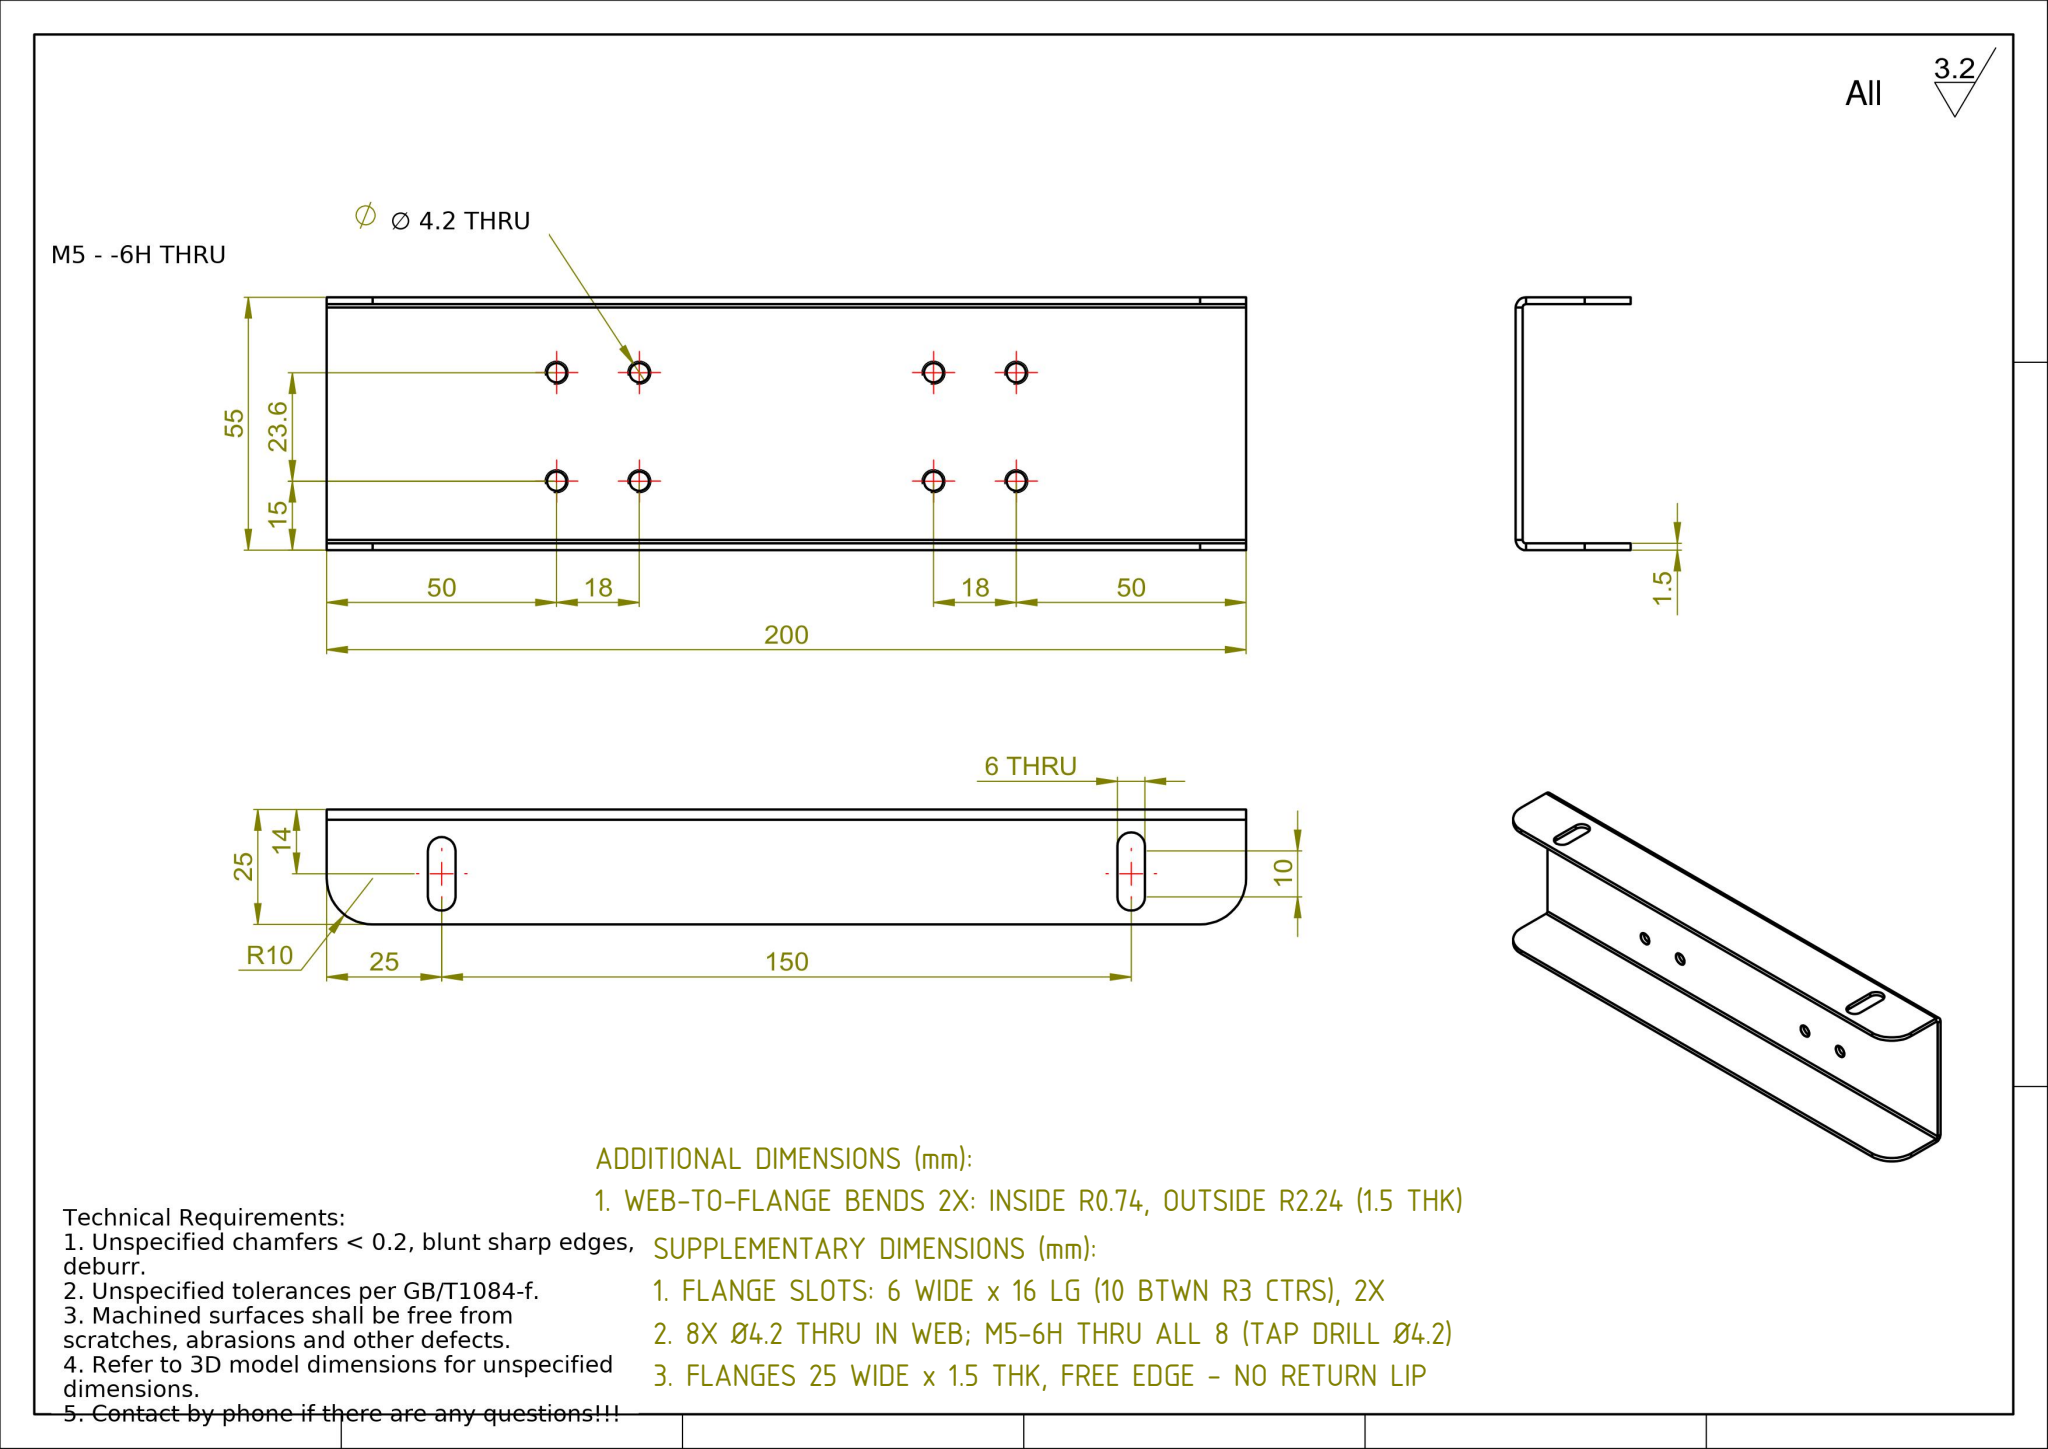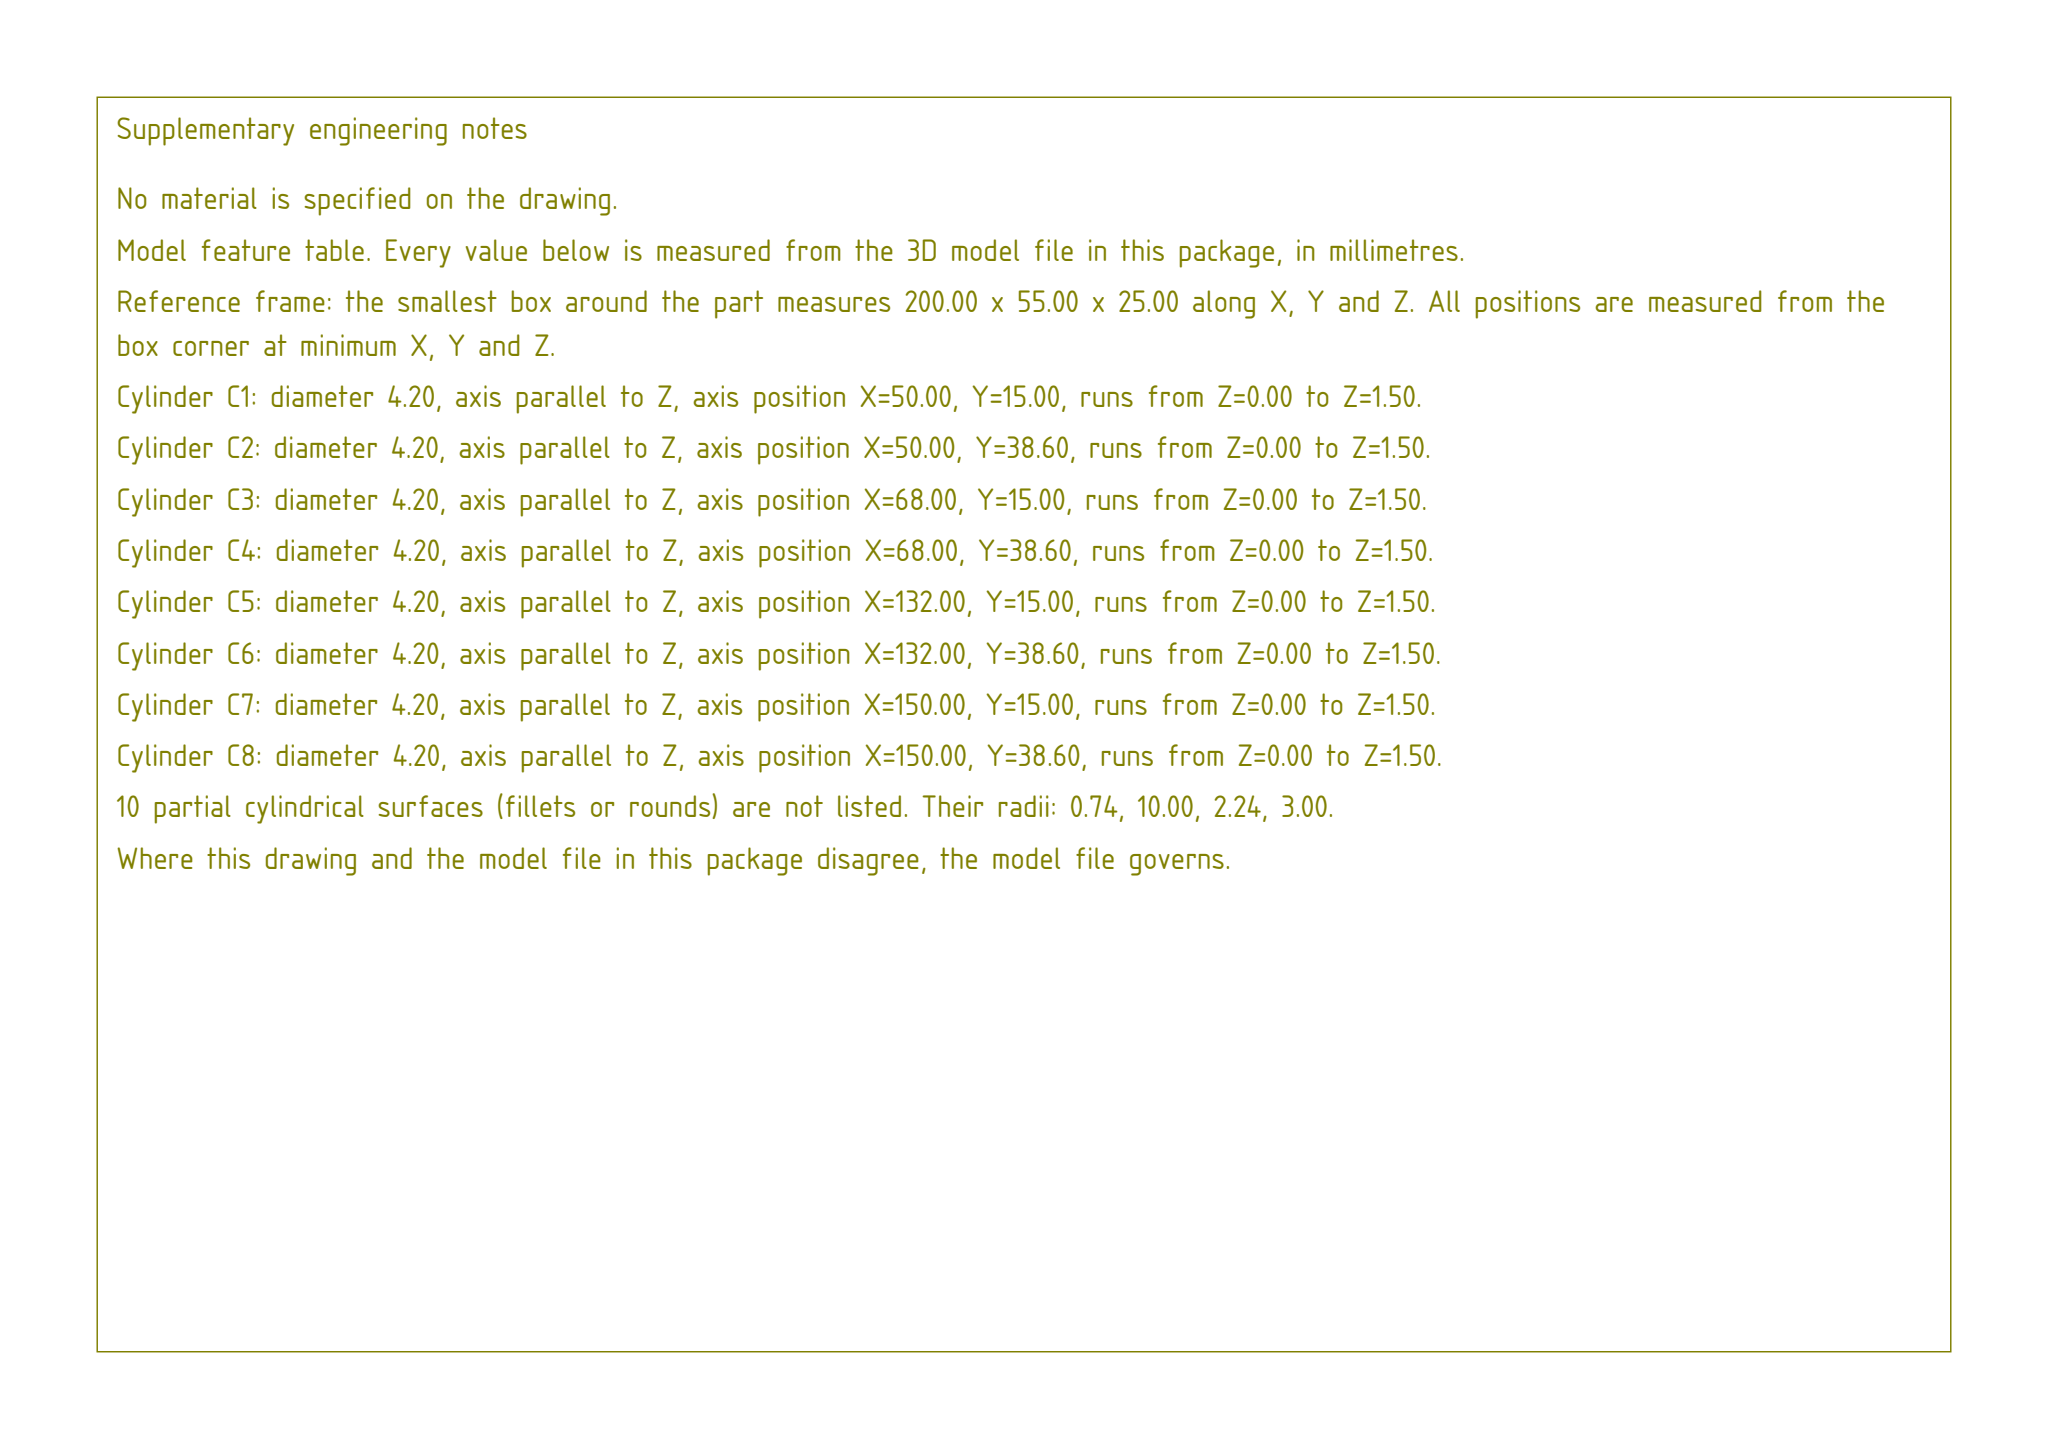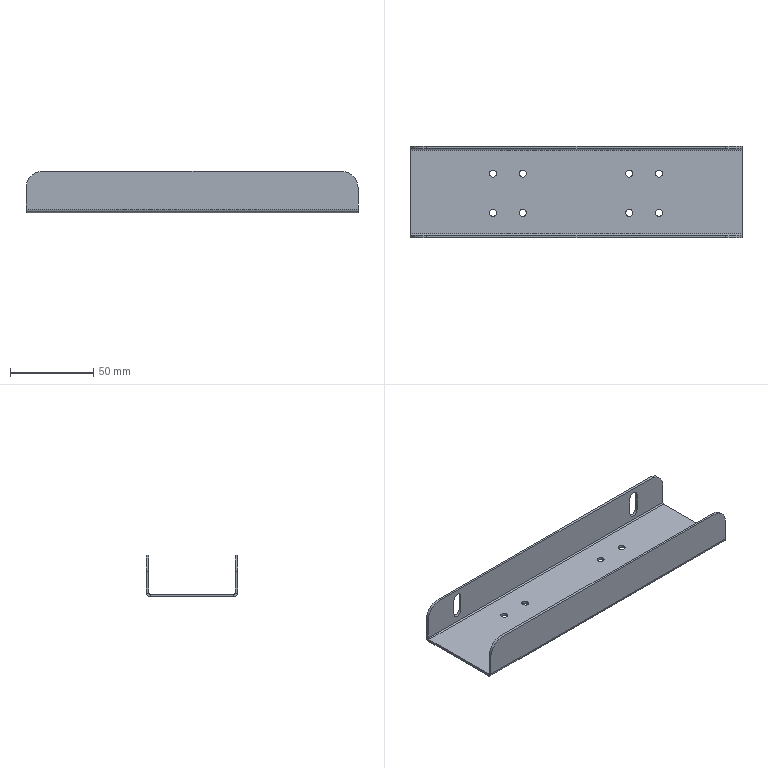Part | SolidWorks | mm | 1 solid | 52 faces | box 200 x 55 x 25 mm | volume 29648 mm3 | cylinder 30 | plane 22 | commonest cylinder face diameters 4.2 x16 6 x6 20 x4 4.473 x2 1.473 x2